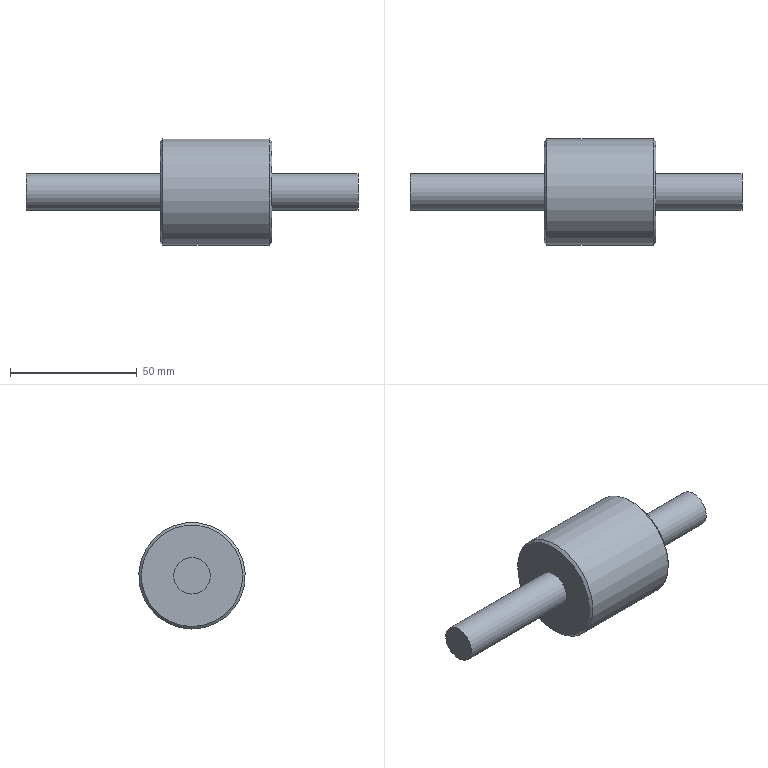Component | NX | 42_LOCATING_PIN | 1 solid | 9 faces | box 131 x 42 x 42 mm | volume 74952 mm3 | plane 4 | cylinder 3 | cone 2 | commonest cylinder face diameters 14.376 x2 42 x1
STEP:
#1=CARTESIAN_POINT('',(0.,0.,0.));
#2=DIRECTION('',(0.,0.,1.));
#3=DIRECTION('',(1.,0.,0.));
#4=AXIS2_PLACEMENT_3D('',#1,#2,#3);
#5=CARTESIAN_POINT('',(53.,-147.739,-31.));
#6=VERTEX_POINT('',#5);
#7=CARTESIAN_POINT('',(53.,-147.739,-10.));
#8=DIRECTION('',(-1.,0.,0.));
#9=DIRECTION('',(0.,0.,-1.));
#10=AXIS2_PLACEMENT_3D('',#7,#8,#9);
#11=CIRCLE('',#10,21.);
#12=CARTESIAN_POINT('',(54.,-147.739,-10.));
#13=DIRECTION('',(-1.,0.,0.));
#14=DIRECTION('',(0.,0.,1.));
#15=AXIS2_PLACEMENT_3D('',#12,#13,#14);
#16=CYLINDRICAL_SURFACE('',#15,21.);
#17=CARTESIAN_POINT('',(3.142,1.));
#18=DIRECTION('',(1.,0.));
#19=VECTOR('',#18,1.);
#20=LINE('',#17,#19);
#21=(GEOMETRIC_REPRESENTATION_CONTEXT(2)PARAMETRIC_REPRESENTATION_CONTEXT()REPRESENTATION_CONTEXT('',''));
#22=DEFINITIONAL_REPRESENTATION('',(#20),#21);
#23=PCURVE('',#16,#22);
#24=CARTESIAN_POINT('',(54.,-147.739,-10.));
#25=DIRECTION('',(-1.,0.,0.));
#26=DIRECTION('',(0.,0.,1.));
#27=AXIS2_PLACEMENT_3D('',#24,#25,#26);
#28=CONICAL_SURFACE('',#27,20.,0.7854);
#29=CARTESIAN_POINT('',(3.142,1.));
#30=DIRECTION('',(1.,0.));
#31=VECTOR('',#30,1.);
#32=LINE('',#29,#31);
#33=(GEOMETRIC_REPRESENTATION_CONTEXT(2)PARAMETRIC_REPRESENTATION_CONTEXT()REPRESENTATION_CONTEXT('',''));
#34=DEFINITIONAL_REPRESENTATION('',(#32),#33);
#35=PCURVE('',#28,#34);
#36=SURFACE_CURVE('',#11,(#23,#35),.PCURVE_S1.);
#37=EDGE_CURVE('',#6,#6,#36,.T.);
#38=ORIENTED_EDGE('',*,*,#37,.T.);
#39=CARTESIAN_POINT('',(11.,-147.739,-31.));
#40=VERTEX_POINT('',#39);
#41=CARTESIAN_POINT('',(53.,-147.739,-31.));
#42=CARTESIAN_POINT('',(11.,-147.739,-31.));
#43=B_SPLINE_CURVE_WITH_KNOTS('',1,(#41,#42),.UNSPECIFIED.,.F.,.F.,(2,2),(1.,43.),.PIECEWISE_BEZIER_KNOTS.);
#44=CARTESIAN_POINT('',(9.425,0.));
#45=DIRECTION('',(0.,1.));
#46=VECTOR('',#45,1.);
#47=LINE('',#44,#46);
#48=(GEOMETRIC_REPRESENTATION_CONTEXT(2)PARAMETRIC_REPRESENTATION_CONTEXT()REPRESENTATION_CONTEXT('',''));
#49=DEFINITIONAL_REPRESENTATION('',(#47),#48);
#50=PCURVE('',#16,#49);
#51=CARTESIAN_POINT('',(3.142,0.));
#52=DIRECTION('',(0.,1.));
#53=VECTOR('',#52,1.);
#54=LINE('',#51,#53);
#55=(GEOMETRIC_REPRESENTATION_CONTEXT(2)PARAMETRIC_REPRESENTATION_CONTEXT()REPRESENTATION_CONTEXT('',''));
#56=DEFINITIONAL_REPRESENTATION('',(#54),#55);
#57=PCURVE('',#16,#56);
#58=SEAM_CURVE('',#43,(#50,#57),.PCURVE_S1.);
#59=EDGE_CURVE('',#6,#40,#58,.T.);
#60=ORIENTED_EDGE('',*,*,#59,.T.);
#61=CARTESIAN_POINT('',(11.,-147.739,-10.));
#62=DIRECTION('',(1.,0.,0.));
#63=DIRECTION('',(0.,0.,-1.));
#64=AXIS2_PLACEMENT_3D('',#61,#62,#63);
#65=CIRCLE('',#64,21.);
#66=CARTESIAN_POINT('',(9.425,43.));
#67=DIRECTION('',(-1.,0.));
#68=VECTOR('',#67,1.);
#69=LINE('',#66,#68);
#70=(GEOMETRIC_REPRESENTATION_CONTEXT(2)PARAMETRIC_REPRESENTATION_CONTEXT()REPRESENTATION_CONTEXT('',''));
#71=DEFINITIONAL_REPRESENTATION('',(#69),#70);
#72=PCURVE('',#16,#71);
#73=CARTESIAN_POINT('',(11.,-147.739,-10.));
#74=DIRECTION('',(1.,0.,0.));
#75=DIRECTION('',(0.,0.,-1.));
#76=AXIS2_PLACEMENT_3D('',#73,#74,#75);
#77=CONICAL_SURFACE('',#76,21.,0.7854);
#78=CARTESIAN_POINT('',(0.,0.));
#79=DIRECTION('',(1.,0.));
#80=VECTOR('',#79,1.);
#81=LINE('',#78,#80);
#82=(GEOMETRIC_REPRESENTATION_CONTEXT(2)PARAMETRIC_REPRESENTATION_CONTEXT()REPRESENTATION_CONTEXT('',''));
#83=DEFINITIONAL_REPRESENTATION('',(#81),#82);
#84=PCURVE('',#77,#83);
#85=SURFACE_CURVE('',#65,(#72,#84),.PCURVE_S1.);
#86=EDGE_CURVE('',#40,#40,#85,.T.);
#87=ORIENTED_EDGE('',*,*,#86,.T.);
#88=ORIENTED_EDGE('',*,*,#59,.F.);
#89=EDGE_LOOP('',(#38,#60,#87,#88));
#90=FACE_BOUND('',#89,.T.);
#91=ADVANCED_FACE('',(#90),#16,.T.);
#92=CARTESIAN_POINT('',(54.,-147.739,-30.));
#93=VERTEX_POINT('',#92);
#94=CARTESIAN_POINT('',(54.,-147.739,-10.));
#95=DIRECTION('',(1.,0.,0.));
#96=DIRECTION('',(0.,0.,-1.));
#97=AXIS2_PLACEMENT_3D('',#94,#95,#96);
#98=CIRCLE('',#97,20.);
#99=CARTESIAN_POINT('',(54.,-147.739,-10.));
#100=DIRECTION('',(1.,0.,0.));
#101=DIRECTION('',(0.,0.,-1.));
#102=AXIS2_PLACEMENT_3D('',#99,#100,#101);
#103=PLANE('',#102);
#104=CARTESIAN_POINT('',(0.,0.));
#105=DIRECTION('',(1.,0.));
#106=AXIS2_PLACEMENT_2D('',#104,#105);
#107=CIRCLE('',#106,20.);
#108=(GEOMETRIC_REPRESENTATION_CONTEXT(2)PARAMETRIC_REPRESENTATION_CONTEXT()REPRESENTATION_CONTEXT('',''));
#109=DEFINITIONAL_REPRESENTATION('',(#107),#108);
#110=PCURVE('',#103,#109);
#111=CARTESIAN_POINT('',(9.425,0.));
#112=DIRECTION('',(-1.,0.));
#113=VECTOR('',#112,1.);
#114=LINE('',#111,#113);
#115=(GEOMETRIC_REPRESENTATION_CONTEXT(2)PARAMETRIC_REPRESENTATION_CONTEXT()REPRESENTATION_CONTEXT('',''));
#116=DEFINITIONAL_REPRESENTATION('',(#114),#115);
#117=PCURVE('',#28,#116);
#118=SURFACE_CURVE('',#98,(#110,#117),.PCURVE_S1.);
#119=EDGE_CURVE('',#93,#93,#118,.T.);
#120=ORIENTED_EDGE('',*,*,#119,.T.);
#121=EDGE_LOOP('',(#120));
#122=FACE_BOUND('',#121,.T.);
#123=CARTESIAN_POINT('',(54.,-147.739,-17.188));
#124=VERTEX_POINT('',#123);
#125=CARTESIAN_POINT('',(54.,-147.739,-10.));
#126=DIRECTION('',(-1.,0.,0.));
#127=DIRECTION('',(0.,0.,-1.));
#128=AXIS2_PLACEMENT_3D('',#125,#126,#127);
#129=CIRCLE('',#128,7.188);
#130=CARTESIAN_POINT('',(7.188,0.));
#131=CARTESIAN_POINT('',(7.188,-12.45));
#132=CARTESIAN_POINT('',(-3.594,-6.225));
#133=CARTESIAN_POINT('',(-14.376,-0.));
#134=CARTESIAN_POINT('',(-3.594,6.225));
#135=CARTESIAN_POINT('',(7.188,12.45));
#136=CARTESIAN_POINT('',(7.188,0.));
#137=(BOUNDED_CURVE()B_SPLINE_CURVE(2,(#130,#131,#132,#133,#134,#135,#136),.UNSPECIFIED.,.T.,.F.)B_SPLINE_CURVE_WITH_KNOTS((1,2,2,2,2,1),(-2.094,0.,2.094,4.189,6.283,8.378),.UNSPECIFIED.)CURVE()GEOMETRIC_REPRESENTATION_ITEM()RATIONAL_B_SPLINE_CURVE((1.,0.5,1.,0.5,1.,0.5,1.))REPRESENTATION_ITEM(''));
#138=(GEOMETRIC_REPRESENTATION_CONTEXT(2)PARAMETRIC_REPRESENTATION_CONTEXT()REPRESENTATION_CONTEXT('',''));
#139=DEFINITIONAL_REPRESENTATION('',(#137),#138);
#140=PCURVE('',#103,#139);
#141=CARTESIAN_POINT('',(78.,-147.739,-10.));
#142=DIRECTION('',(-1.,0.,0.));
#143=DIRECTION('',(0.,0.,1.));
#144=AXIS2_PLACEMENT_3D('',#141,#142,#143);
#145=CYLINDRICAL_SURFACE('',#144,7.188);
#146=CARTESIAN_POINT('',(3.142,24.));
#147=DIRECTION('',(1.,0.));
#148=VECTOR('',#147,1.);
#149=LINE('',#146,#148);
#150=(GEOMETRIC_REPRESENTATION_CONTEXT(2)PARAMETRIC_REPRESENTATION_CONTEXT()REPRESENTATION_CONTEXT('',''));
#151=DEFINITIONAL_REPRESENTATION('',(#149),#150);
#152=PCURVE('',#145,#151);
#153=SURFACE_CURVE('',#129,(#140,#152),.PCURVE_S1.);
#154=EDGE_CURVE('',#124,#124,#153,.T.);
#155=ORIENTED_EDGE('',*,*,#154,.T.);
#156=EDGE_LOOP('',(#155));
#157=FACE_BOUND('',#156,.T.);
#158=ADVANCED_FACE('',(#122,#157),#103,.T.);
#159=CARTESIAN_POINT('',(10.,-147.739,-30.));
#160=VERTEX_POINT('',#159);
#161=CARTESIAN_POINT('',(10.,-147.739,-10.));
#162=DIRECTION('',(-1.,0.,0.));
#163=DIRECTION('',(0.,0.,-1.));
#164=AXIS2_PLACEMENT_3D('',#161,#162,#163);
#165=CIRCLE('',#164,20.);
#166=CARTESIAN_POINT('',(10.,-147.739,-10.));
#167=DIRECTION('',(1.,0.,0.));
#168=DIRECTION('',(0.,0.,-1.));
#169=AXIS2_PLACEMENT_3D('',#166,#167,#168);
#170=PLANE('',#169);
#171=CARTESIAN_POINT('',(20.,0.));
#172=CARTESIAN_POINT('',(20.,-34.641));
#173=CARTESIAN_POINT('',(-10.,-17.321));
#174=CARTESIAN_POINT('',(-40.,-0.));
#175=CARTESIAN_POINT('',(-10.,17.321));
#176=CARTESIAN_POINT('',(20.,34.641));
#177=CARTESIAN_POINT('',(20.,0.));
#178=(BOUNDED_CURVE()B_SPLINE_CURVE(2,(#171,#172,#173,#174,#175,#176,#177),.UNSPECIFIED.,.T.,.F.)B_SPLINE_CURVE_WITH_KNOTS((1,2,2,2,2,1),(-2.094,0.,2.094,4.189,6.283,8.378),.UNSPECIFIED.)CURVE()GEOMETRIC_REPRESENTATION_ITEM()RATIONAL_B_SPLINE_CURVE((1.,0.5,1.,0.5,1.,0.5,1.))REPRESENTATION_ITEM(''));
#179=(GEOMETRIC_REPRESENTATION_CONTEXT(2)PARAMETRIC_REPRESENTATION_CONTEXT()REPRESENTATION_CONTEXT('',''));
#180=DEFINITIONAL_REPRESENTATION('',(#178),#179);
#181=PCURVE('',#170,#180);
#182=CARTESIAN_POINT('',(6.283,-1.));
#183=DIRECTION('',(-1.,0.));
#184=VECTOR('',#183,1.);
#185=LINE('',#182,#184);
#186=(GEOMETRIC_REPRESENTATION_CONTEXT(2)PARAMETRIC_REPRESENTATION_CONTEXT()REPRESENTATION_CONTEXT('',''));
#187=DEFINITIONAL_REPRESENTATION('',(#185),#186);
#188=PCURVE('',#77,#187);
#189=SURFACE_CURVE('',#165,(#181,#188),.PCURVE_S1.);
#190=EDGE_CURVE('',#160,#160,#189,.T.);
#191=ORIENTED_EDGE('',*,*,#190,.T.);
#192=EDGE_LOOP('',(#191));
#193=FACE_BOUND('',#192,.T.);
#194=CARTESIAN_POINT('',(10.,-147.739,-17.188));
#195=VERTEX_POINT('',#194);
#196=CARTESIAN_POINT('',(10.,-147.739,-10.));
#197=DIRECTION('',(-1.,0.,0.));
#198=DIRECTION('',(0.,0.,-1.));
#199=AXIS2_PLACEMENT_3D('',#196,#197,#198);
#200=CIRCLE('',#199,7.188);
#201=CARTESIAN_POINT('',(7.188,0.));
#202=CARTESIAN_POINT('',(7.188,-12.45));
#203=CARTESIAN_POINT('',(-3.594,-6.225));
#204=CARTESIAN_POINT('',(-14.376,-0.));
#205=CARTESIAN_POINT('',(-3.594,6.225));
#206=CARTESIAN_POINT('',(7.188,12.45));
#207=CARTESIAN_POINT('',(7.188,0.));
#208=(BOUNDED_CURVE()B_SPLINE_CURVE(2,(#201,#202,#203,#204,#205,#206,#207),.UNSPECIFIED.,.T.,.F.)B_SPLINE_CURVE_WITH_KNOTS((1,2,2,2,2,1),(-2.094,0.,2.094,4.189,6.283,8.378),.UNSPECIFIED.)CURVE()GEOMETRIC_REPRESENTATION_ITEM()RATIONAL_B_SPLINE_CURVE((1.,0.5,1.,0.5,1.,0.5,1.))REPRESENTATION_ITEM(''));
#209=(GEOMETRIC_REPRESENTATION_CONTEXT(2)PARAMETRIC_REPRESENTATION_CONTEXT()REPRESENTATION_CONTEXT('',''));
#210=DEFINITIONAL_REPRESENTATION('',(#208),#209);
#211=PCURVE('',#170,#210);
#212=CARTESIAN_POINT('',(78.,-147.739,-10.));
#213=DIRECTION('',(-1.,0.,0.));
#214=DIRECTION('',(0.,0.,1.));
#215=AXIS2_PLACEMENT_3D('',#212,#213,#214);
#216=CYLINDRICAL_SURFACE('',#215,7.188);
#217=CARTESIAN_POINT('',(3.142,68.));
#218=DIRECTION('',(1.,0.));
#219=VECTOR('',#218,1.);
#220=LINE('',#217,#219);
#221=(GEOMETRIC_REPRESENTATION_CONTEXT(2)PARAMETRIC_REPRESENTATION_CONTEXT()REPRESENTATION_CONTEXT('',''));
#222=DEFINITIONAL_REPRESENTATION('',(#220),#221);
#223=PCURVE('',#216,#222);
#224=SURFACE_CURVE('',#200,(#211,#223),.PCURVE_S1.);
#225=EDGE_CURVE('',#195,#195,#224,.T.);
#226=ORIENTED_EDGE('',*,*,#225,.F.);
#227=EDGE_LOOP('',(#226));
#228=FACE_BOUND('',#227,.T.);
#229=ADVANCED_FACE('',(#193,#228),#170,.F.);
#230=CARTESIAN_POINT('',(-43.,-147.739,-17.188));
#231=VERTEX_POINT('',#230);
#232=CARTESIAN_POINT('',(-43.,-147.739,-10.));
#233=DIRECTION('',(1.,0.,0.));
#234=DIRECTION('',(0.,0.,-1.));
#235=AXIS2_PLACEMENT_3D('',#232,#233,#234);
#236=CIRCLE('',#235,7.188);
#237=CARTESIAN_POINT('',(-43.,-147.739,-10.));
#238=DIRECTION('',(1.,0.,0.));
#239=DIRECTION('',(0.,0.,-1.));
#240=AXIS2_PLACEMENT_3D('',#237,#238,#239);
#241=PLANE('',#240);
#242=CARTESIAN_POINT('',(0.,0.));
#243=DIRECTION('',(1.,0.));
#244=AXIS2_PLACEMENT_2D('',#242,#243);
#245=CIRCLE('',#244,7.188);
#246=(GEOMETRIC_REPRESENTATION_CONTEXT(2)PARAMETRIC_REPRESENTATION_CONTEXT()REPRESENTATION_CONTEXT('',''));
#247=DEFINITIONAL_REPRESENTATION('',(#245),#246);
#248=PCURVE('',#241,#247);
#249=CARTESIAN_POINT('',(9.425,121.));
#250=DIRECTION('',(-1.,0.));
#251=VECTOR('',#250,1.);
#252=LINE('',#249,#251);
#253=(GEOMETRIC_REPRESENTATION_CONTEXT(2)PARAMETRIC_REPRESENTATION_CONTEXT()REPRESENTATION_CONTEXT('',''));
#254=DEFINITIONAL_REPRESENTATION('',(#252),#253);
#255=PCURVE('',#216,#254);
#256=SURFACE_CURVE('',#236,(#248,#255),.PCURVE_S1.);
#257=EDGE_CURVE('',#231,#231,#256,.T.);
#258=ORIENTED_EDGE('',*,*,#257,.F.);
#259=EDGE_LOOP('',(#258));
#260=FACE_BOUND('',#259,.T.);
#261=ADVANCED_FACE('',(#260),#241,.F.);
#262=ORIENTED_EDGE('',*,*,#257,.T.);
#263=CARTESIAN_POINT('',(10.,-147.739,-17.188));
#264=CARTESIAN_POINT('',(-43.,-147.739,-17.188));
#265=B_SPLINE_CURVE_WITH_KNOTS('',1,(#263,#264),.UNSPECIFIED.,.F.,.F.,(2,2),(68.,121.),.PIECEWISE_BEZIER_KNOTS.);
#266=CARTESIAN_POINT('',(3.142,0.));
#267=DIRECTION('',(0.,1.));
#268=VECTOR('',#267,1.);
#269=LINE('',#266,#268);
#270=(GEOMETRIC_REPRESENTATION_CONTEXT(2)PARAMETRIC_REPRESENTATION_CONTEXT()REPRESENTATION_CONTEXT('',''));
#271=DEFINITIONAL_REPRESENTATION('',(#269),#270);
#272=PCURVE('',#216,#271);
#273=CARTESIAN_POINT('',(9.425,0.));
#274=DIRECTION('',(0.,1.));
#275=VECTOR('',#274,1.);
#276=LINE('',#273,#275);
#277=(GEOMETRIC_REPRESENTATION_CONTEXT(2)PARAMETRIC_REPRESENTATION_CONTEXT()REPRESENTATION_CONTEXT('',''));
#278=DEFINITIONAL_REPRESENTATION('',(#276),#277);
#279=PCURVE('',#216,#278);
#280=SEAM_CURVE('',#265,(#272,#279),.PCURVE_S1.);
#281=EDGE_CURVE('',#195,#231,#280,.T.);
#282=ORIENTED_EDGE('',*,*,#281,.F.);
#283=ORIENTED_EDGE('',*,*,#225,.T.);
#284=ORIENTED_EDGE('',*,*,#281,.T.);
#285=EDGE_LOOP('',(#262,#282,#283,#284));
#286=FACE_BOUND('',#285,.T.);
#287=ADVANCED_FACE('',(#286),#216,.T.);
#288=ORIENTED_EDGE('',*,*,#154,.F.);
#289=CARTESIAN_POINT('',(88.,-147.739,-17.188));
#290=VERTEX_POINT('',#289);
#291=CARTESIAN_POINT('',(88.,-147.739,-17.188));
#292=CARTESIAN_POINT('',(54.,-147.739,-17.188));
#293=B_SPLINE_CURVE_WITH_KNOTS('',1,(#291,#292),.UNSPECIFIED.,.F.,.F.,(2,2),(-10.,24.),.PIECEWISE_BEZIER_KNOTS.);
#294=CARTESIAN_POINT('',(3.142,0.));
#295=DIRECTION('',(0.,1.));
#296=VECTOR('',#295,1.);
#297=LINE('',#294,#296);
#298=(GEOMETRIC_REPRESENTATION_CONTEXT(2)PARAMETRIC_REPRESENTATION_CONTEXT()REPRESENTATION_CONTEXT('',''));
#299=DEFINITIONAL_REPRESENTATION('',(#297),#298);
#300=PCURVE('',#145,#299);
#301=CARTESIAN_POINT('',(9.425,0.));
#302=DIRECTION('',(0.,1.));
#303=VECTOR('',#302,1.);
#304=LINE('',#301,#303);
#305=(GEOMETRIC_REPRESENTATION_CONTEXT(2)PARAMETRIC_REPRESENTATION_CONTEXT()REPRESENTATION_CONTEXT('',''));
#306=DEFINITIONAL_REPRESENTATION('',(#304),#305);
#307=PCURVE('',#145,#306);
#308=SEAM_CURVE('',#293,(#300,#307),.PCURVE_S1.);
#309=EDGE_CURVE('',#290,#124,#308,.T.);
#310=ORIENTED_EDGE('',*,*,#309,.F.);
#311=CARTESIAN_POINT('',(88.,-147.739,-10.));
#312=DIRECTION('',(1.,0.,0.));
#313=DIRECTION('',(0.,0.,-1.));
#314=AXIS2_PLACEMENT_3D('',#311,#312,#313);
#315=CIRCLE('',#314,7.188);
#316=CARTESIAN_POINT('',(9.425,-10.));
#317=DIRECTION('',(-1.,0.));
#318=VECTOR('',#317,1.);
#319=LINE('',#316,#318);
#320=(GEOMETRIC_REPRESENTATION_CONTEXT(2)PARAMETRIC_REPRESENTATION_CONTEXT()REPRESENTATION_CONTEXT('',''));
#321=DEFINITIONAL_REPRESENTATION('',(#319),#320);
#322=PCURVE('',#145,#321);
#323=CARTESIAN_POINT('',(88.,-147.739,-10.));
#324=DIRECTION('',(1.,0.,0.));
#325=DIRECTION('',(0.,0.,-1.));
#326=AXIS2_PLACEMENT_3D('',#323,#324,#325);
#327=PLANE('',#326);
#328=CARTESIAN_POINT('',(0.,0.));
#329=DIRECTION('',(1.,0.));
#330=AXIS2_PLACEMENT_2D('',#328,#329);
#331=CIRCLE('',#330,7.188);
#332=(GEOMETRIC_REPRESENTATION_CONTEXT(2)PARAMETRIC_REPRESENTATION_CONTEXT()REPRESENTATION_CONTEXT('',''));
#333=DEFINITIONAL_REPRESENTATION('',(#331),#332);
#334=PCURVE('',#327,#333);
#335=SURFACE_CURVE('',#315,(#322,#334),.PCURVE_S1.);
#336=EDGE_CURVE('',#290,#290,#335,.T.);
#337=ORIENTED_EDGE('',*,*,#336,.F.);
#338=ORIENTED_EDGE('',*,*,#309,.T.);
#339=EDGE_LOOP('',(#288,#310,#337,#338));
#340=FACE_BOUND('',#339,.T.);
#341=ADVANCED_FACE('',(#340),#145,.T.);
#342=ORIENTED_EDGE('',*,*,#336,.T.);
#343=EDGE_LOOP('',(#342));
#344=FACE_BOUND('',#343,.T.);
#345=ADVANCED_FACE('',(#344),#327,.T.);
#346=ORIENTED_EDGE('',*,*,#37,.F.);
#347=CARTESIAN_POINT('',(54.,-147.739,-30.));
#348=CARTESIAN_POINT('',(53.,-147.739,-31.));
#349=B_SPLINE_CURVE_WITH_KNOTS('',1,(#347,#348),.UNSPECIFIED.,.F.,.F.,(2,2),(0.,1.414),.PIECEWISE_BEZIER_KNOTS.);
#350=CARTESIAN_POINT('',(3.142,0.));
#351=DIRECTION('',(0.,1.));
#352=VECTOR('',#351,1.);
#353=LINE('',#350,#352);
#354=(GEOMETRIC_REPRESENTATION_CONTEXT(2)PARAMETRIC_REPRESENTATION_CONTEXT()REPRESENTATION_CONTEXT('',''));
#355=DEFINITIONAL_REPRESENTATION('',(#353),#354);
#356=PCURVE('',#28,#355);
#357=CARTESIAN_POINT('',(9.425,0.));
#358=DIRECTION('',(0.,1.));
#359=VECTOR('',#358,1.);
#360=LINE('',#357,#359);
#361=(GEOMETRIC_REPRESENTATION_CONTEXT(2)PARAMETRIC_REPRESENTATION_CONTEXT()REPRESENTATION_CONTEXT('',''));
#362=DEFINITIONAL_REPRESENTATION('',(#360),#361);
#363=PCURVE('',#28,#362);
#364=SEAM_CURVE('',#349,(#356,#363),.PCURVE_S1.);
#365=EDGE_CURVE('',#93,#6,#364,.T.);
#366=ORIENTED_EDGE('',*,*,#365,.F.);
#367=ORIENTED_EDGE('',*,*,#119,.F.);
#368=ORIENTED_EDGE('',*,*,#365,.T.);
#369=EDGE_LOOP('',(#346,#366,#367,#368));
#370=FACE_BOUND('',#369,.T.);
#371=ADVANCED_FACE('',(#370),#28,.T.);
#372=ORIENTED_EDGE('',*,*,#190,.F.);
#373=CARTESIAN_POINT('',(10.,-147.739,-30.));
#374=CARTESIAN_POINT('',(11.,-147.739,-31.));
#375=B_SPLINE_CURVE_WITH_KNOTS('',1,(#373,#374),.UNSPECIFIED.,.F.,.F.,(2,2),(-1.414,0.),.PIECEWISE_BEZIER_KNOTS.);
#376=CARTESIAN_POINT('',(6.283,0.));
#377=DIRECTION('',(0.,1.));
#378=VECTOR('',#377,1.);
#379=LINE('',#376,#378);
#380=(GEOMETRIC_REPRESENTATION_CONTEXT(2)PARAMETRIC_REPRESENTATION_CONTEXT()REPRESENTATION_CONTEXT('',''));
#381=DEFINITIONAL_REPRESENTATION('',(#379),#380);
#382=PCURVE('',#77,#381);
#383=CARTESIAN_POINT('',(0.,0.));
#384=DIRECTION('',(0.,1.));
#385=VECTOR('',#384,1.);
#386=LINE('',#383,#385);
#387=(GEOMETRIC_REPRESENTATION_CONTEXT(2)PARAMETRIC_REPRESENTATION_CONTEXT()REPRESENTATION_CONTEXT('',''));
#388=DEFINITIONAL_REPRESENTATION('',(#386),#387);
#389=PCURVE('',#77,#388);
#390=SEAM_CURVE('',#375,(#382,#389),.PCURVE_S1.);
#391=EDGE_CURVE('',#160,#40,#390,.T.);
#392=ORIENTED_EDGE('',*,*,#391,.T.);
#393=ORIENTED_EDGE('',*,*,#86,.F.);
#394=ORIENTED_EDGE('',*,*,#391,.F.);
#395=EDGE_LOOP('',(#372,#392,#393,#394));
#396=FACE_BOUND('',#395,.T.);
#397=ADVANCED_FACE('',(#396),#77,.T.);
#398=CLOSED_SHELL('',(#91,#158,#229,#261,#287,#341,#345,#371,#397));
#399=MANIFOLD_SOLID_BREP('',#398);
#400=(LENGTH_UNIT()NAMED_UNIT(*)SI_UNIT(.MILLI.,.METRE.));
#401=UNCERTAINTY_MEASURE_WITH_UNIT(LENGTH_MEASURE(0.00001),#400,'','');
#402=(NAMED_UNIT(*)PLANE_ANGLE_UNIT()SI_UNIT($,.RADIAN.));
#403=(NAMED_UNIT(*)SI_UNIT($,.STERADIAN.)SOLID_ANGLE_UNIT());
#404=(GEOMETRIC_REPRESENTATION_CONTEXT(3)GLOBAL_UNCERTAINTY_ASSIGNED_CONTEXT((#401))GLOBAL_UNIT_ASSIGNED_CONTEXT((#400,#402,#403))REPRESENTATION_CONTEXT('',''));
#405=ADVANCED_BREP_SHAPE_REPRESENTATION('',(#4,#399),#404);